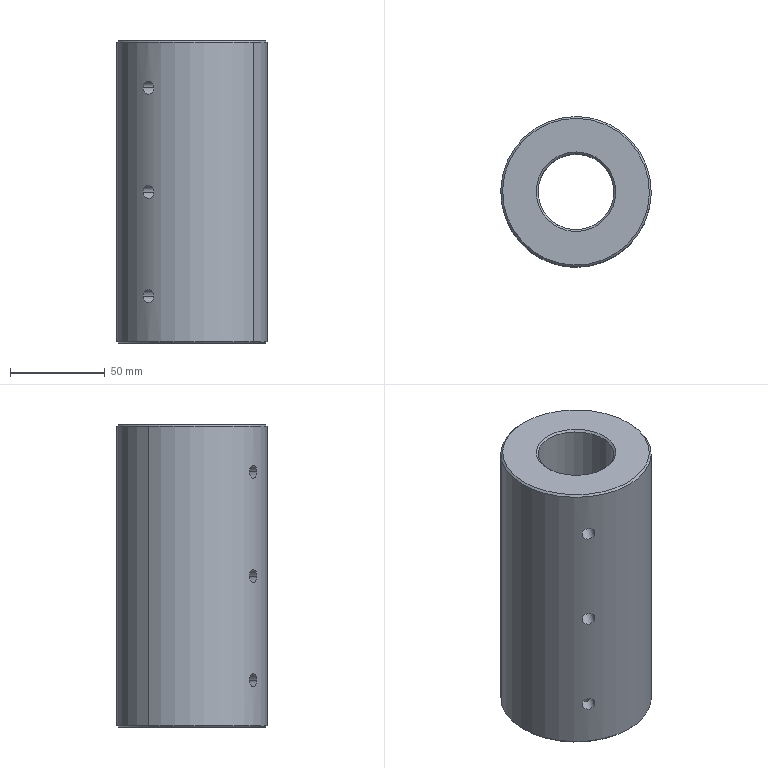Component | SolidWorks | 8TC-A17001-20-06CoreSleeve-1 | 1 solid | 26 faces | box 79.5 x 79.5 x 160 mm | volume 588701 mm3 | cylinder 14 | cone 10 | plane 2 | commonest cylinder face diameters 6.8 x6 5 x4 40.1 x2 79.5 x2 | material #45
build123d program:
from build123d import *

# Parameters (mm, degrees)
SKETCH1_R                  = 39.75
SKETCH1_R_2                = 20.05
BOSS_EXTRUDE1_DEPTH        = 80
M6_TAPPED_HOLE1_D          = 5
M6_TAPPED_HOLE1_DEPTH      = 25
M6_TAPPED_HOLE1_TIP        = 1.502
SKETCH6_W                  = 3.4
SKETCH6_H                  = 39.75
M8_TAPPED_HOLE1_AT_2_COUNT = 2
M8_TAPPED_HOLE1_AT_2_PITCH = 55
M8_TAPPED_HOLE1_AT_3_COUNT = 2
M8_TAPPED_HOLE1_AT_3_PITCH = 110
CHAMFER1_SIZE              = 1


with BuildPart() as part:
    # Sketch1 → Boss-Extrude1 (new, symmetric)
    with BuildSketch(Plane(origin=(0, 0, 0), x_dir=(1, 0, 0), z_dir=(0, 1, 0))):
        with Locations(Location((0, 0, 0), (0, 0, 270))):
            Circle(SKETCH1_R)
        with Locations(Location((0, 0, 0), (0, 0, 270))):
            Circle(SKETCH1_R_2, mode=Mode.SUBTRACT)
    extrude(amount=BOSS_EXTRUDE1_DEPTH, both=True)

    # M6 Tapped Hole1
    with Locations(Plane(origin=(0, 80, 0), x_dir=(1, 0, 0), z_dir=(0, 1, 0))):
        with Locations((30, 0), (-30, 0)):
            Hole(M6_TAPPED_HOLE1_D / 2, depth=M6_TAPPED_HOLE1_DEPTH)
            with Locations((0, 0, -(M6_TAPPED_HOLE1_DEPTH + M6_TAPPED_HOLE1_TIP / 2))):  # 118° drill point
                Cone(0, M6_TAPPED_HOLE1_D / 2, M6_TAPPED_HOLE1_TIP, mode=Mode.SUBTRACT)

    # Sketch6 → M8 Tapped Hole1 (revolve, cut)
    with BuildSketch(Plane.ZX.offset(55)):
        with Locations((1.7, 19.875)):
            Rectangle(SKETCH6_W, SKETCH6_H)
    m8_tapped_hole1 = revolve(axis=Axis((-6.35, 55, 0), (1, 0, 0)), mode=Mode.SUBTRACT)

    # M8 Tapped Hole1 at 2: M8 Tapped Hole1 ×2
    with Locations(*[(0, -i * M8_TAPPED_HOLE1_AT_2_PITCH, 0) for i in range(1, M8_TAPPED_HOLE1_AT_2_COUNT)]):
        add(m8_tapped_hole1, mode=Mode.SUBTRACT)

    # M8 Tapped Hole1 at 3: M8 Tapped Hole1 ×2
    with Locations(*[(0, -i * M8_TAPPED_HOLE1_AT_3_PITCH, 0) for i in range(1, M8_TAPPED_HOLE1_AT_3_COUNT)]):
        add(m8_tapped_hole1, mode=Mode.SUBTRACT)

    # Chamfer1
    chamfer1_edges = [part.edges().sort_by_distance(p)[0] for p in [
        (0, -80, -39.75),
        (0, 80, -39.75),
        (0, -80, -20.05),
        (0, 80, -20.05),
    ]]
    chamfer(chamfer1_edges, length=CHAMFER1_SIZE)


solid = part.part

# Placed as in the assembly
solid = solid.moved(Location((733.029, 200.722, 192.5), (90, 54.528, -180)))